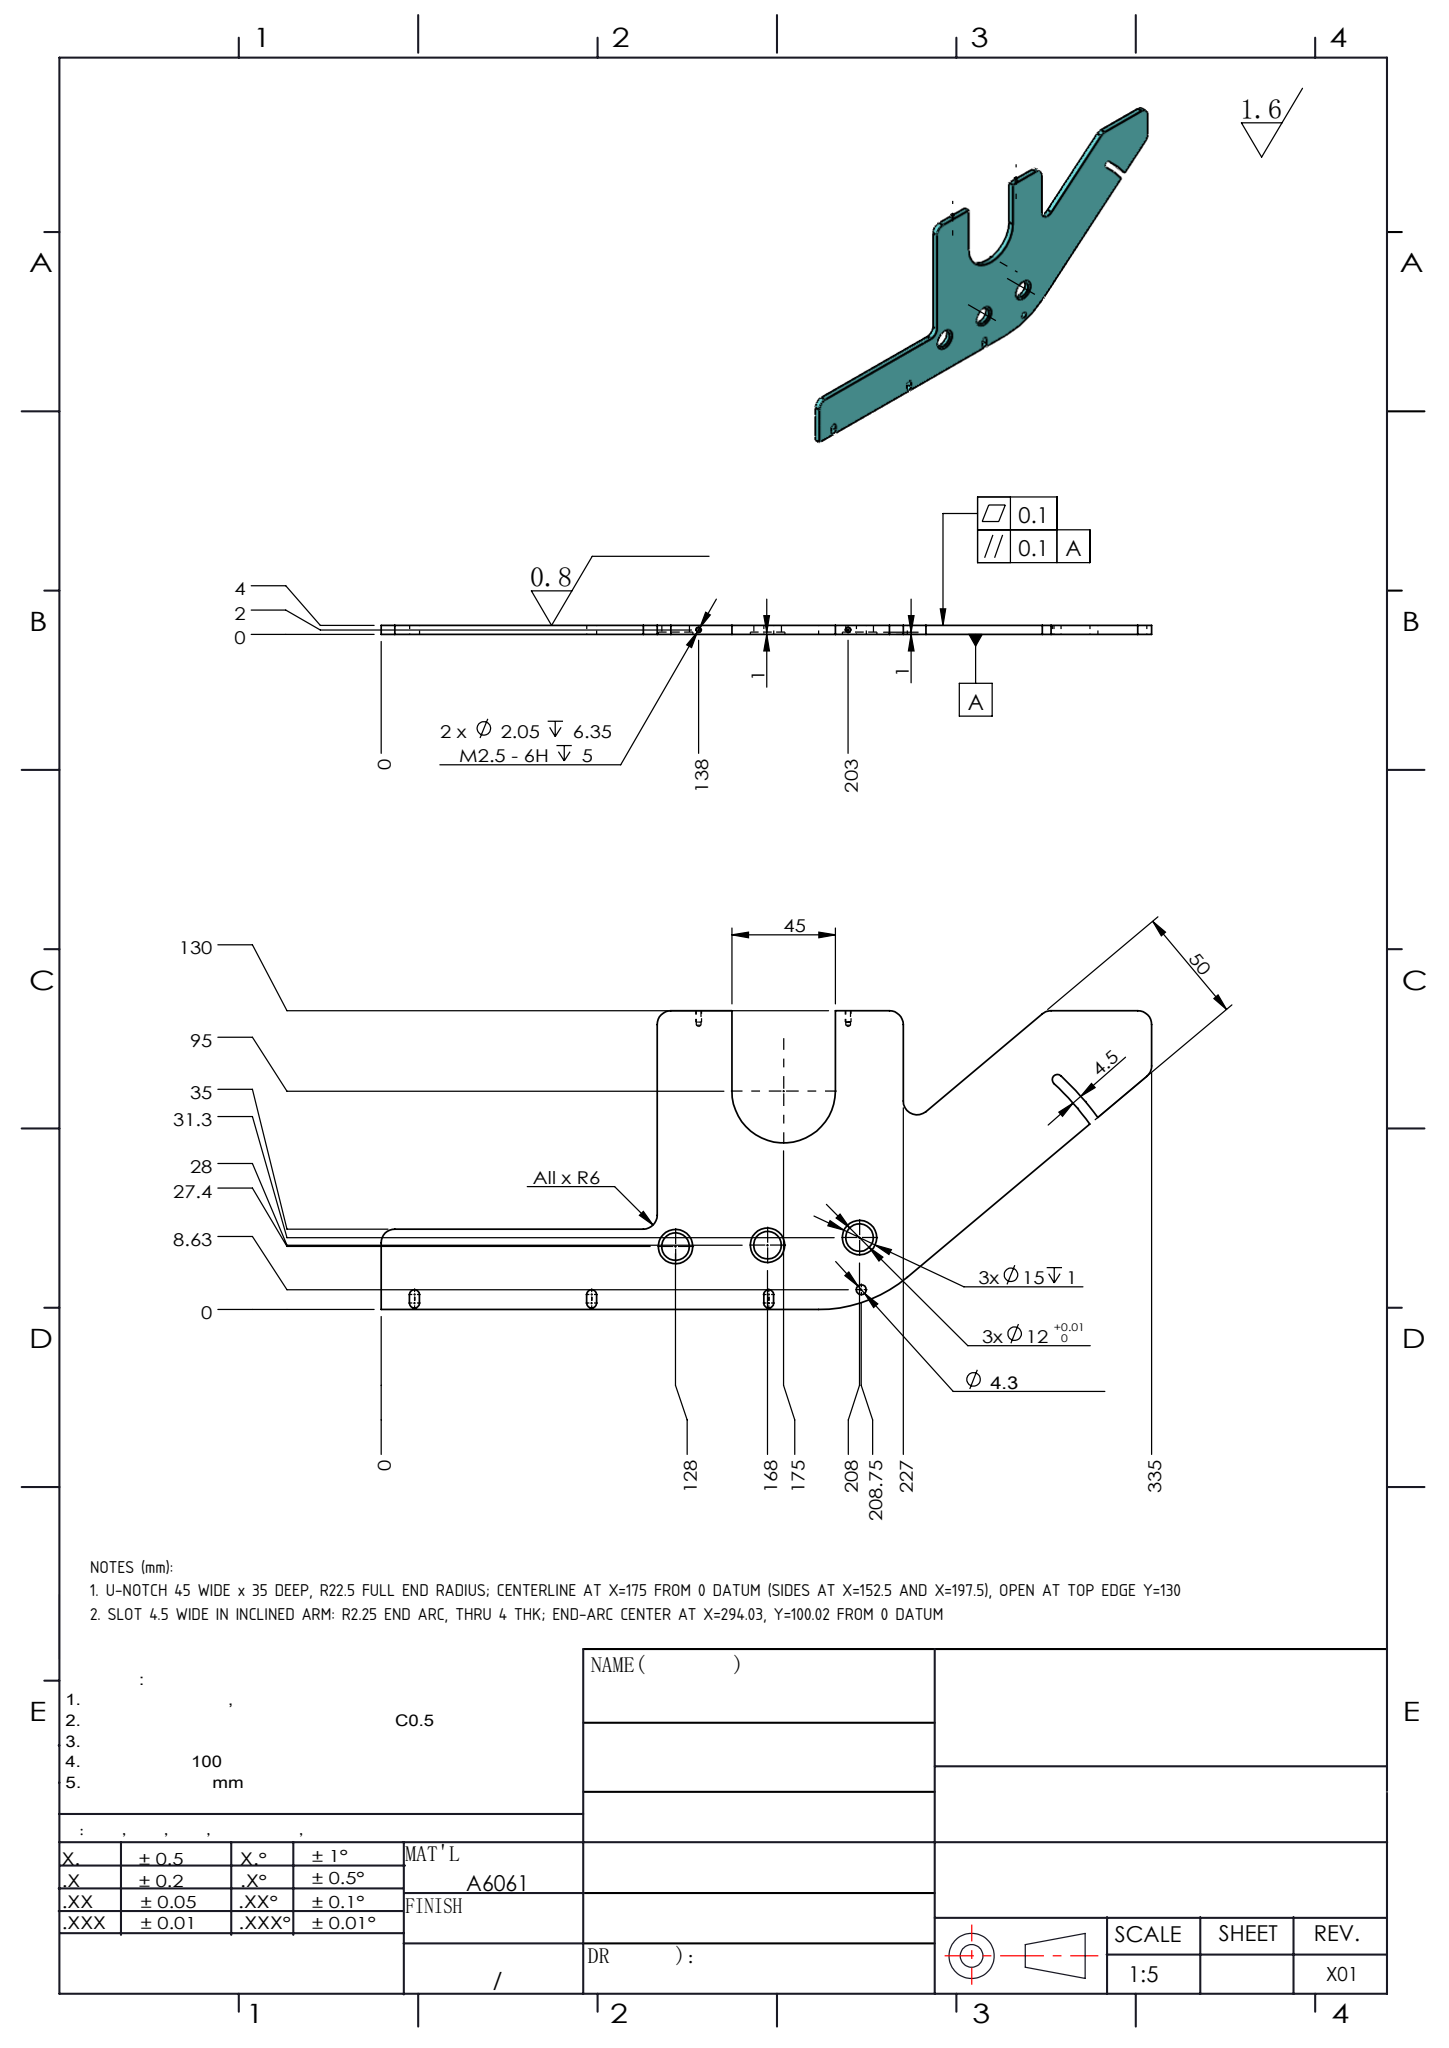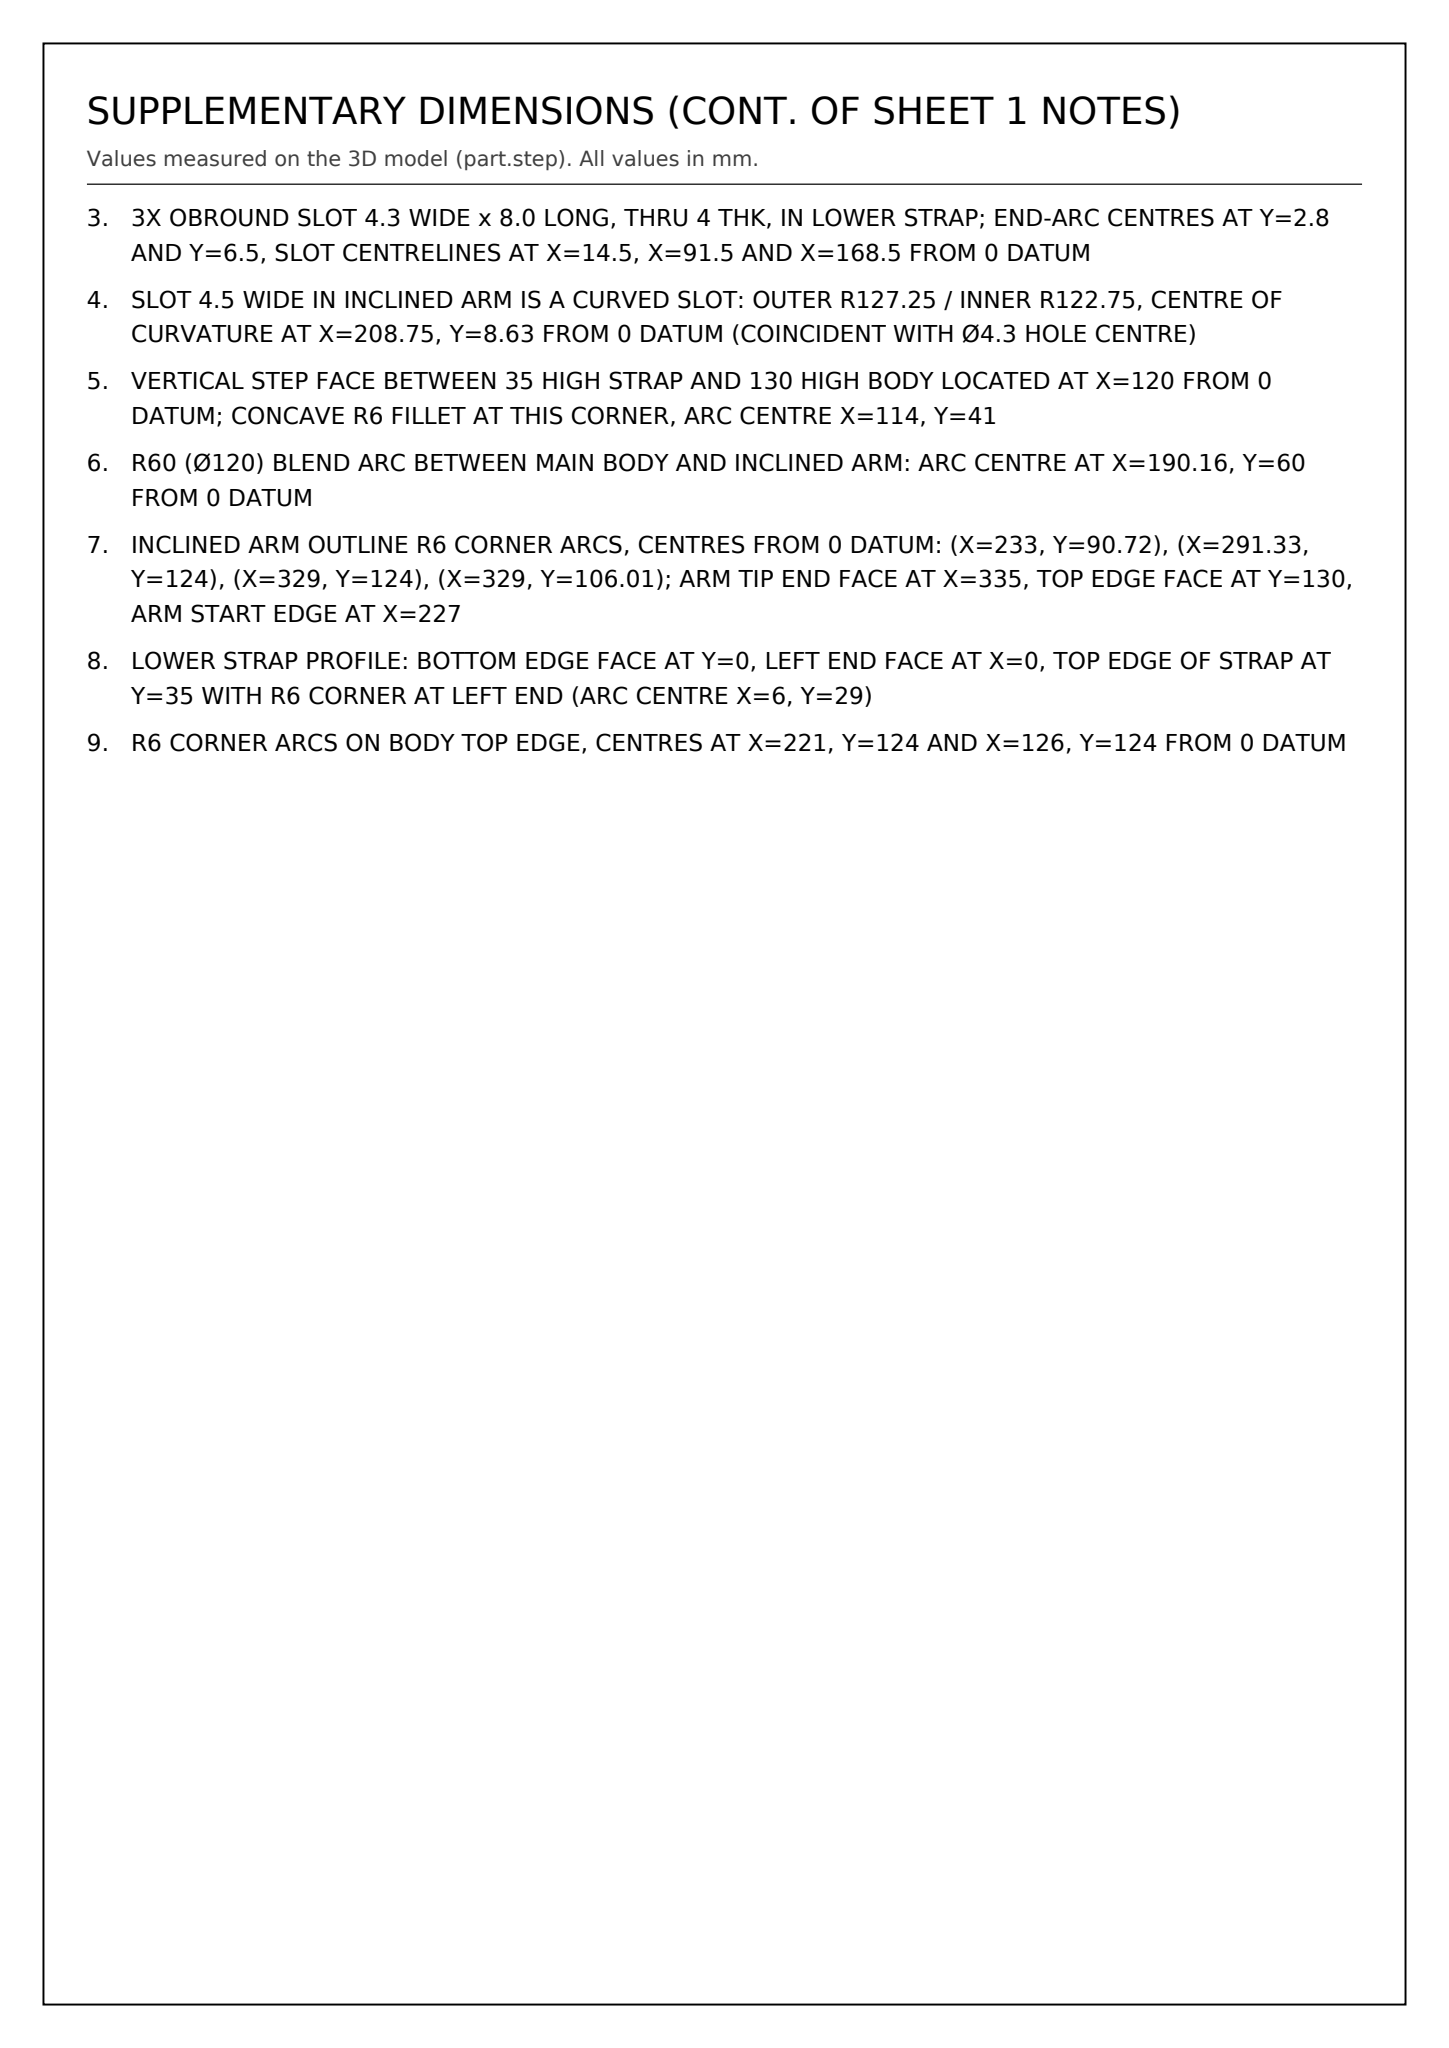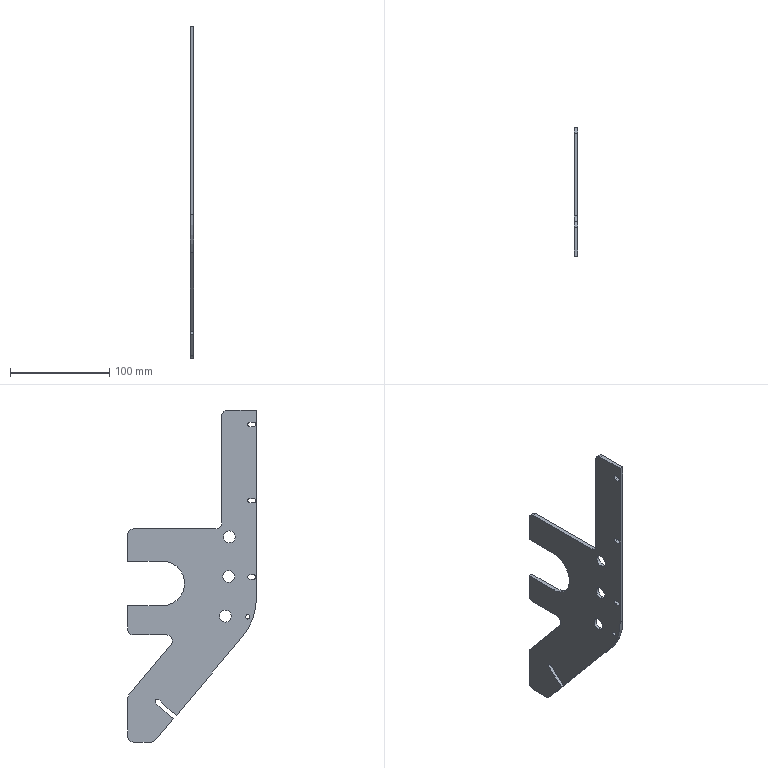Part | SolidWorks | mm | 1 solid | 66 faces | box 4 x 130 x 335 mm | volume 84604 mm3 | cylinder 37 | plane 25 | cone 4 | commonest cylinder face diameters 12 x14 4.3 x8 15 x6 2.05 x4 120 x1 245.5 x1 254.5 x1 4.5 x1
Drawing notes:
U-NOTCH 45 WIDE x 35 DEEP, R22.5 FULL END RADIUS; CENTERLINE AT X=175 FROM 0 DATUM (SIDES AT X=152.5 AND X=197.5), OPEN AT TOP EDGE Y=130 | from the solid: cylinder dia 45, axis x, pos y=95 z=160, length 4 (thru); axis planes z=137.5 and z=182.5; plane y=130 (X = 335 - z)
SLOT 4.5 WIDE IN INCLINED ARM: R2.25 END ARC, THRU 4 THK; END-ARC CENTER AT X=294.03, Y=100.02 FROM 0 DATUM | from the solid: cylinder dia 4.5, axis x, pos y=100.02 z=40.97, length 4 (X = 335 - z)
3X OBROUND SLOT 4.3 WIDE x 8.0 LONG, THRU 4 THK, IN LOWER STRAP; END-ARC CENTRES AT Y=2.8 AND Y=6.5, SLOT CENTRELINES AT X=14.5, X=91.5 AND X=168.5 FROM 0 DATUM | from the solid: Ø4.3 thru-cylinders (len 4 = full thk) at (y=2.8, z=166.5/243.5/320.5) and (y=6.5, z=166.5/243.5/320.5); X=335-z gives 168.5/91.5/14.5; arc-centre spacing 6.5-2.8=3.7 plus 4.3 width = 8.0 overall length, not 7.6
SLOT 4.5 WIDE IN INCLINED ARM IS A CURVED SLOT: OUTER R127.25 / INNER R122.75, CENTRE OF CURVATURE AT X=208.75, Y=8.63 FROM 0 DATUM (COINCIDENT WITH Ø4.3 HOLE CENTRE) | from the solid: cylinders dia 254.5 and 245.5, axis x, at y=8.63, z=126.25 (X=335-126.25=208.75), length 4
VERTICAL STEP FACE BETWEEN 35 HIGH STRAP AND 130 HIGH BODY LOCATED AT X=120 FROM 0 DATUM; CONCAVE R6 FILLET AT THIS CORNER, ARC CENTRE X=114, Y=41 | from the solid: plane normal z at offset 215 (X=335-215=120); cylinder dia 12 axis x at y=41, z=221 (X=114)
R60 (Ø120) BLEND ARC BETWEEN MAIN BODY AND INCLINED ARM: ARC CENTRE AT X=190.16, Y=60 FROM 0 DATUM | from the solid: cylinder dia 120, axis x, at y=60, z=144.84 (X=335-144.84=190.16), length 4
INCLINED ARM OUTLINE R6 CORNER ARCS, CENTRES FROM 0 DATUM: (X=233, Y=90.72), (X=291.33, Y=124), (X=329, Y=124), (X=329, Y=106.01); ARM TIP END FACE AT X=335, TOP EDGE FACE AT Y=130, ARM START EDGE AT X=227 | from the solid: cylinders dia 12 axis x at (y=90.72,z=102), (y=124,z=43.67), (y=124,z=6), (y=106.01,z=6); planes normal z at 0 (X=335) and 108 (X=227); planes normal y at 130
LOWER STRAP PROFILE: BOTTOM EDGE FACE AT Y=0, LEFT END FACE AT X=0, TOP EDGE OF STRAP AT Y=35 WITH R6 CORNER AT LEFT END (ARC CENTRE X=6, Y=29) | from the solid: planes normal y at 0 and 35; plane normal z at 335 (X=0); cylinder dia 12 axis x at y=29, z=329 (X=6)
R6 CORNER ARCS ON BODY TOP EDGE, CENTRES AT X=221, Y=124 AND X=126, Y=124 FROM 0 DATUM | from the solid: cylinders dia 12 axis x at (y=124, z=114) and (y=124, z=209), length 4